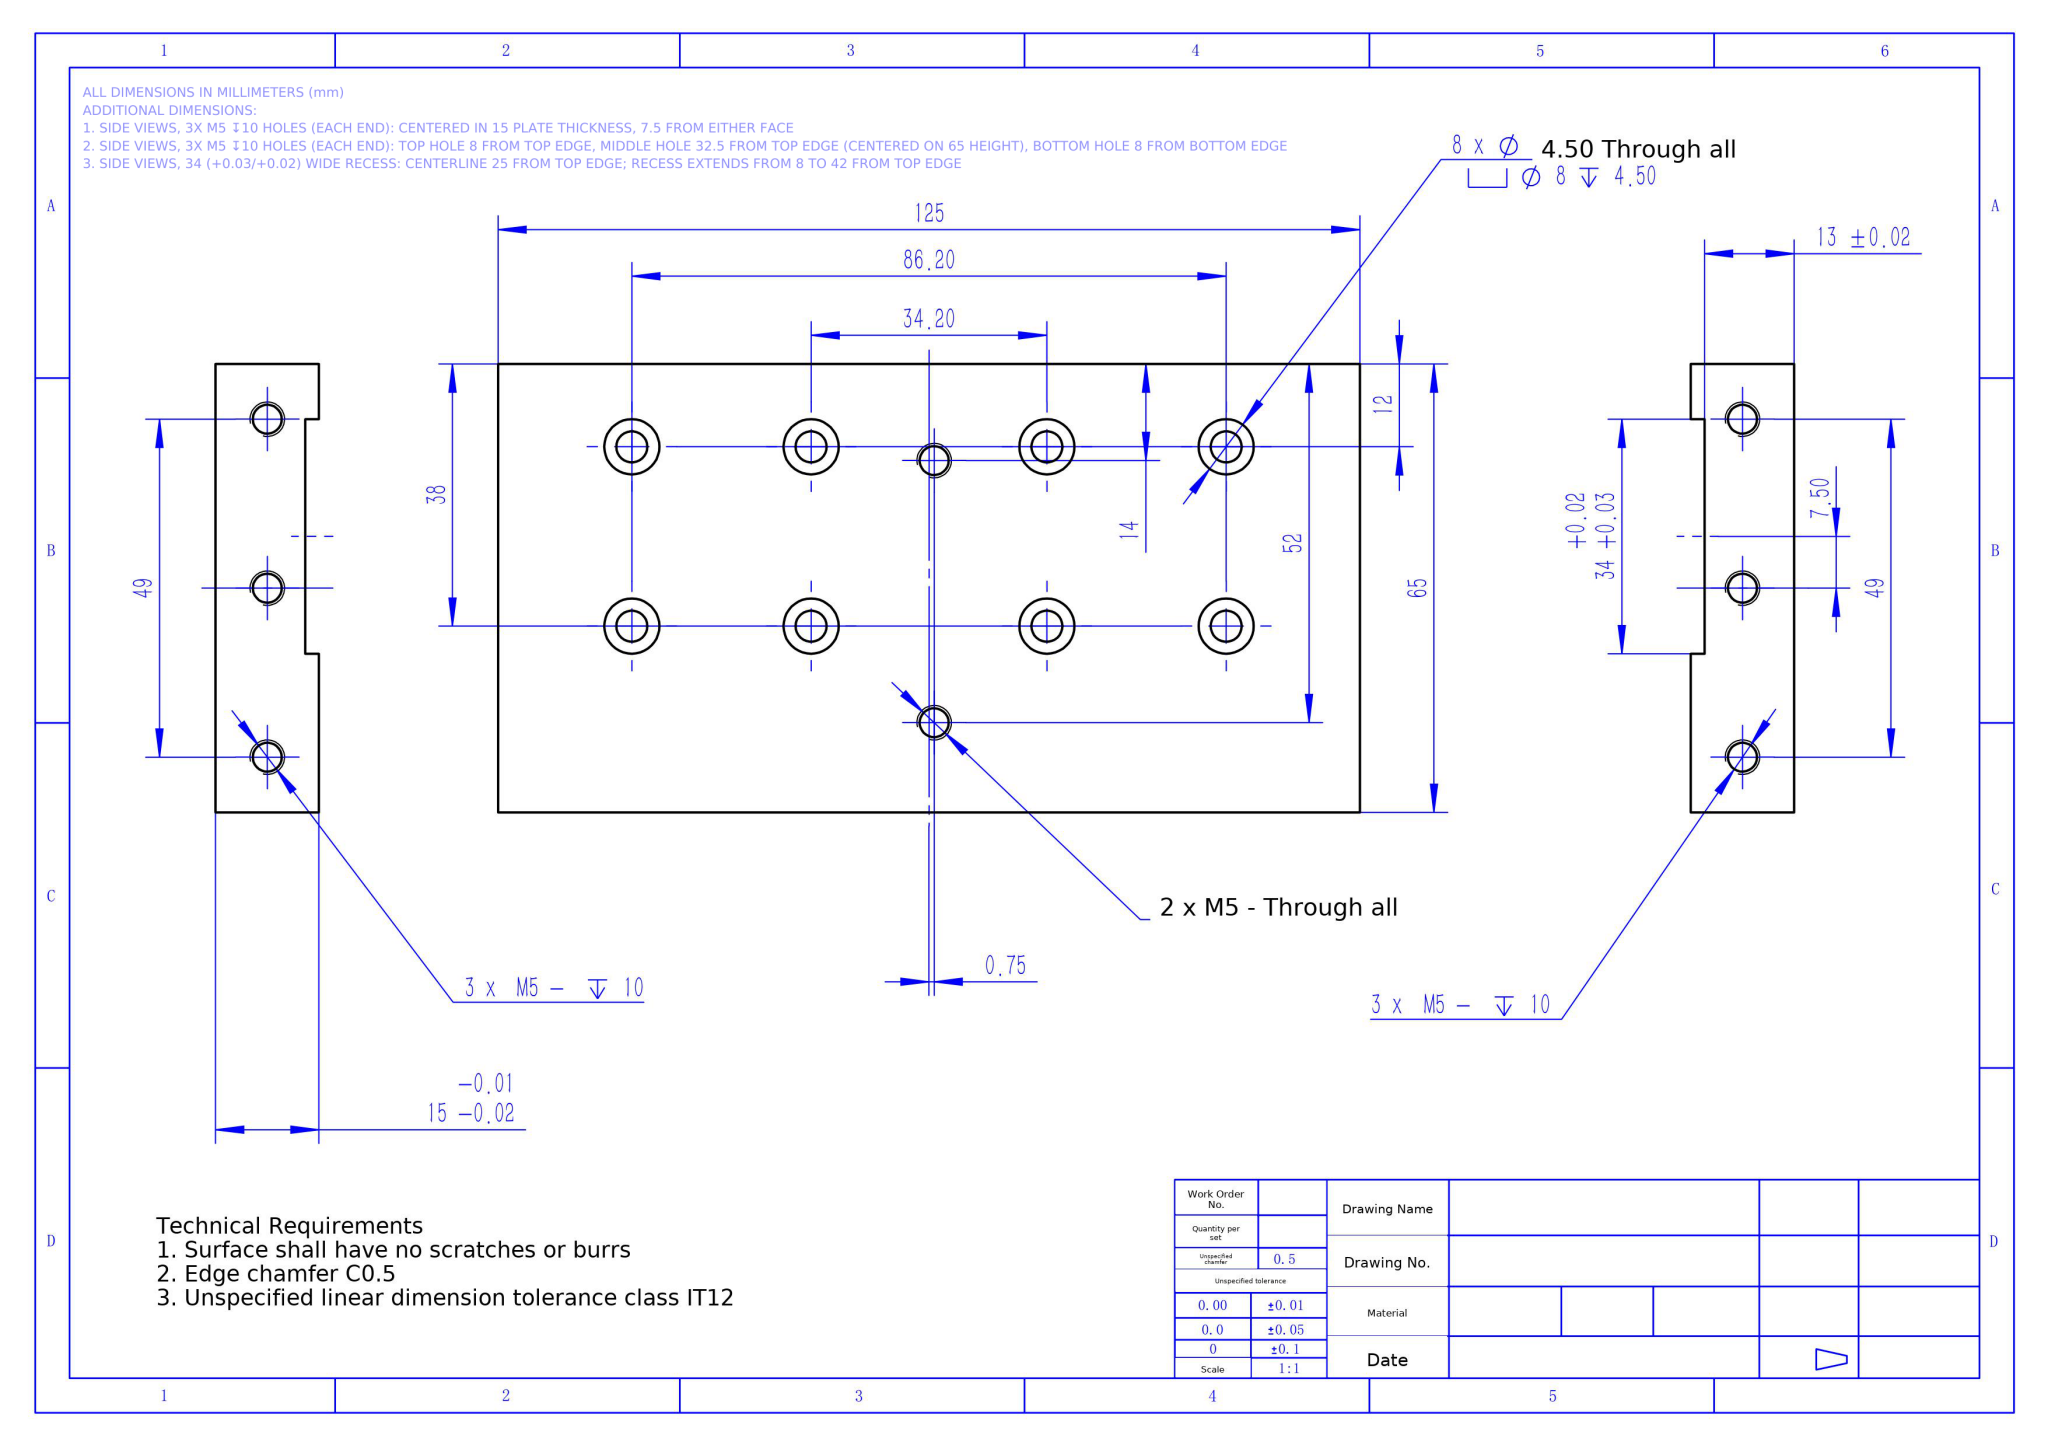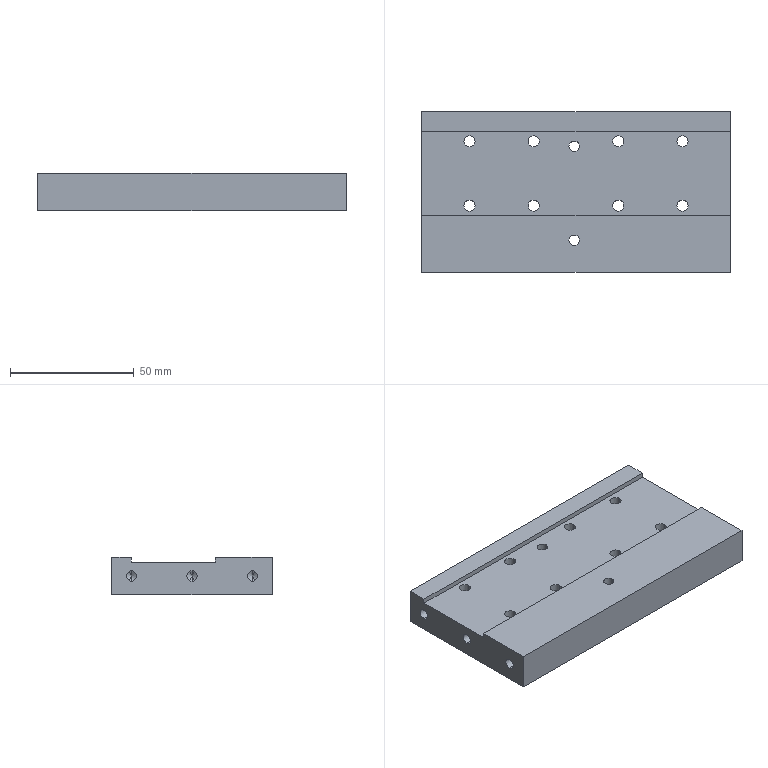Part | NX | mm | 1 solid | 78 faces | box 125 x 65 x 15 mm | volume 109030 mm3 | cylinder 48 | plane 18 | cone 12 | commonest cylinder face diameters 4.2 x16 8 x16 4.5 x16